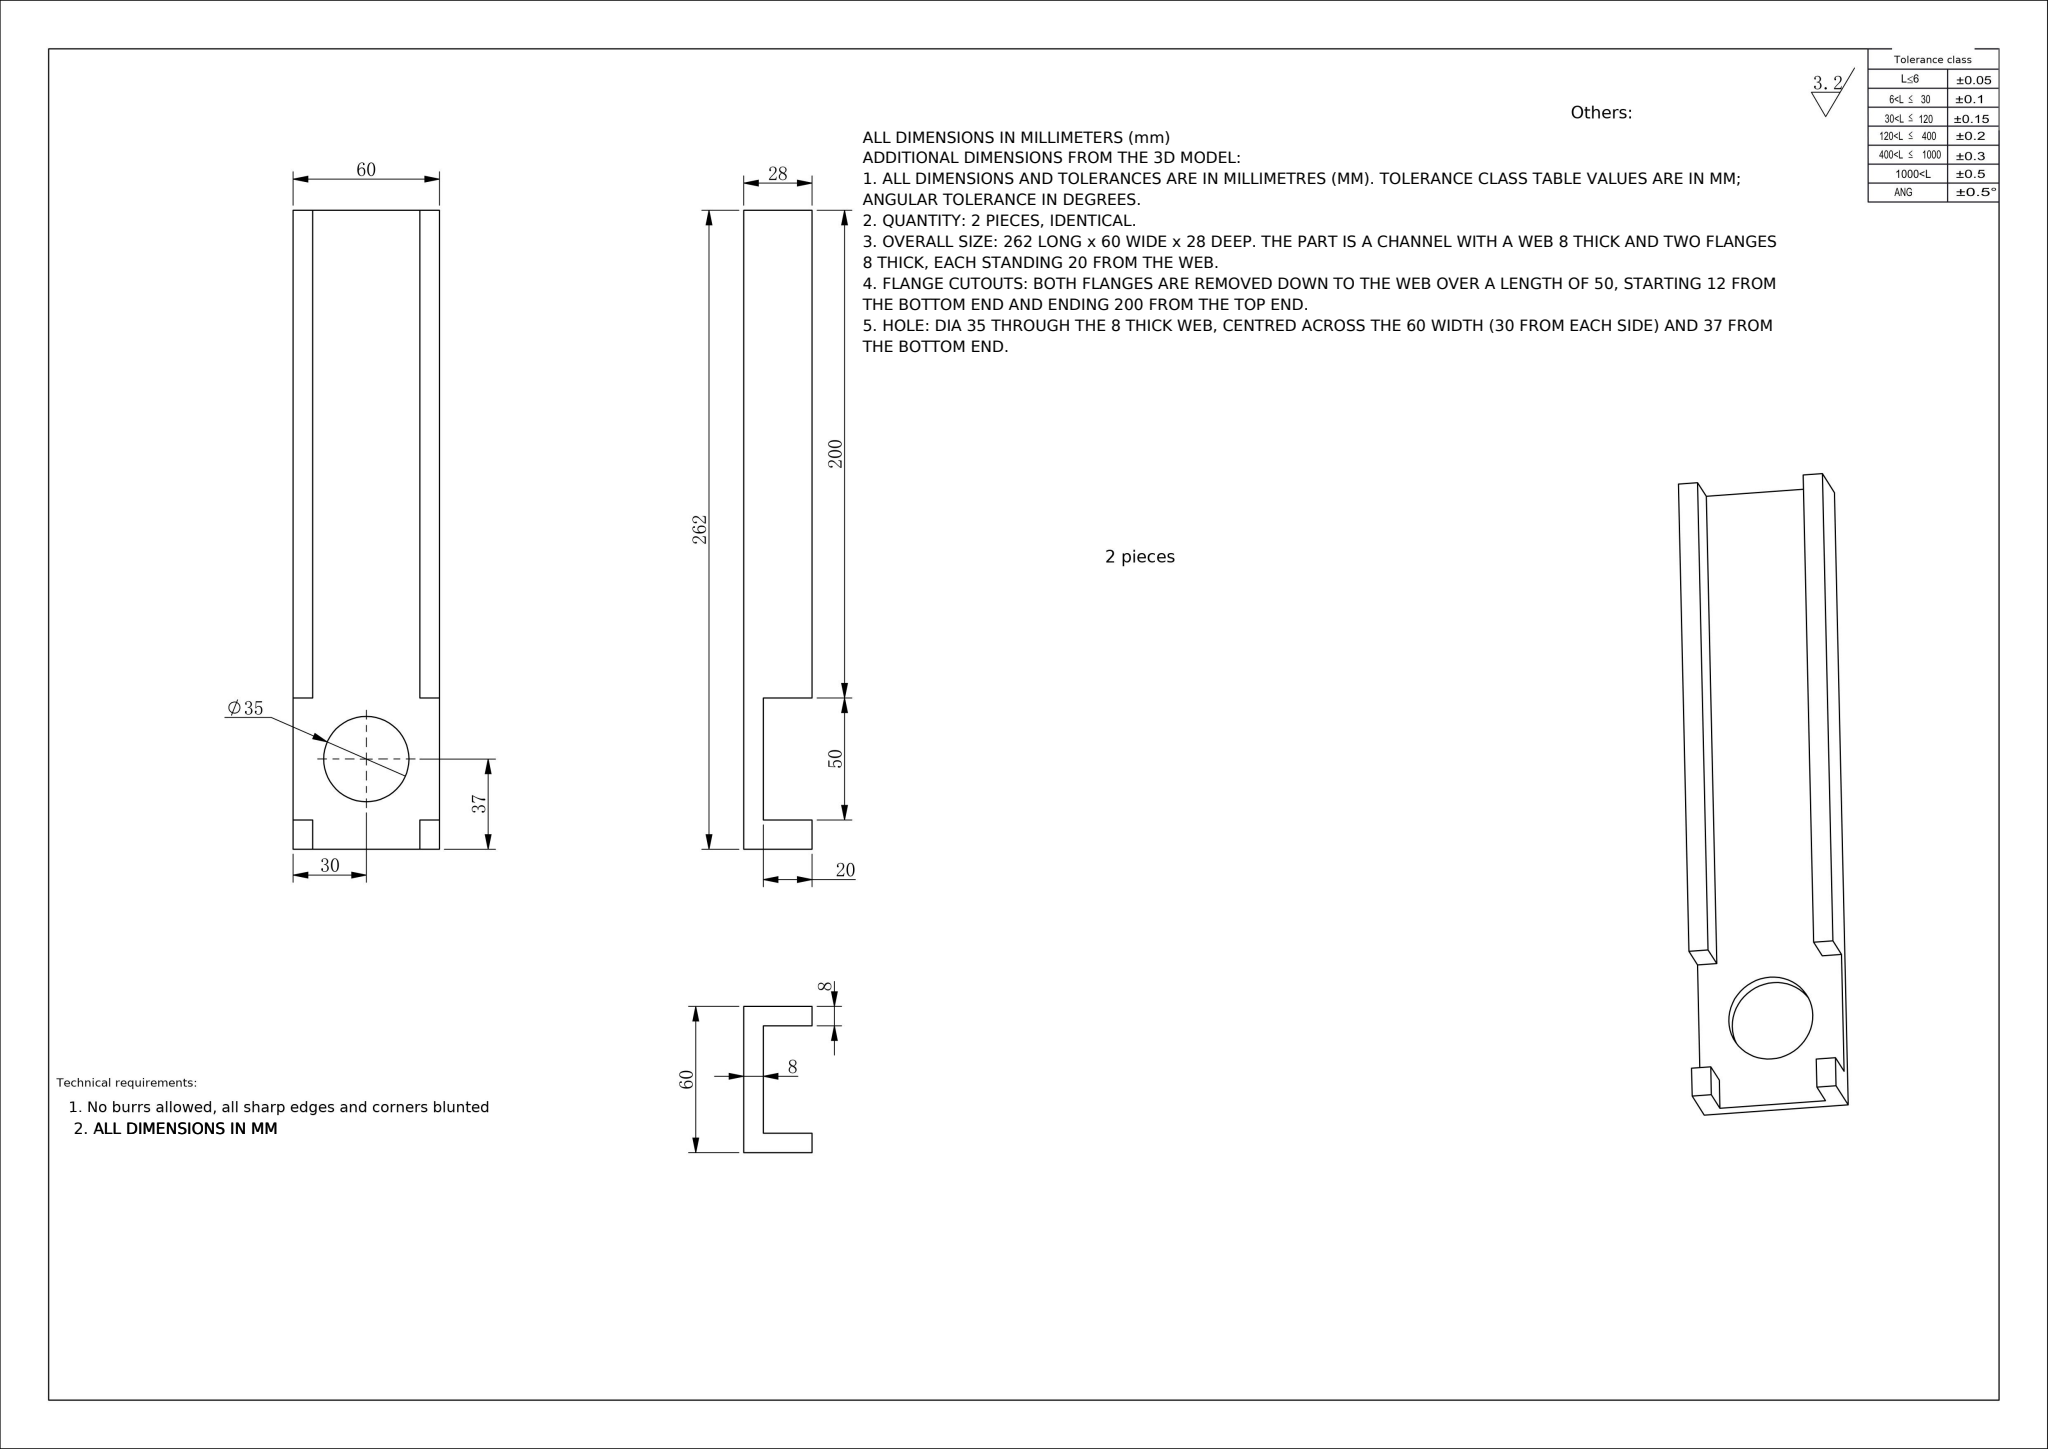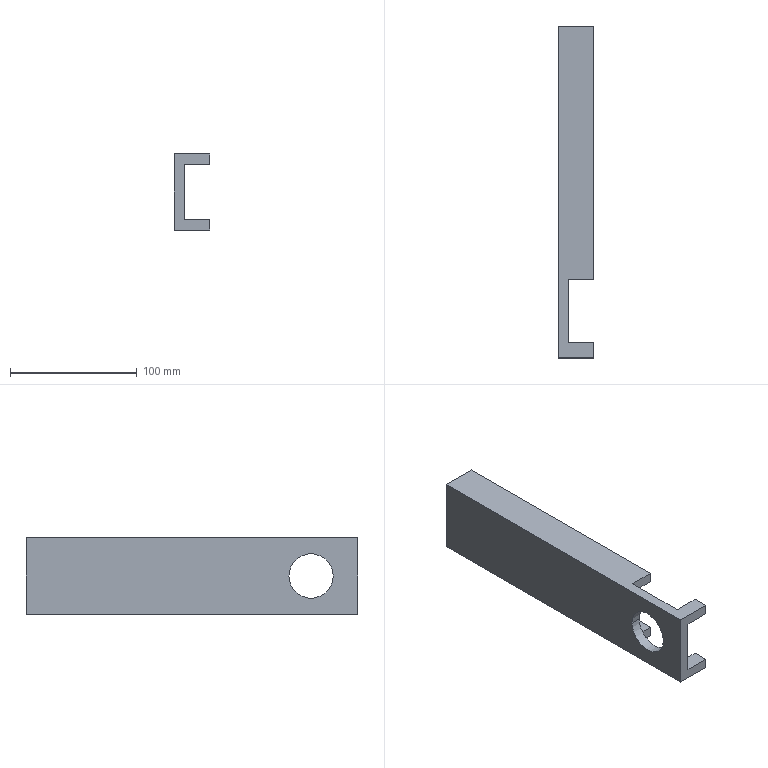Part | NX | mm | Forked Upright Pedestal Bracket | 1 solid | 20 faces | box 28 x 262 x 60 mm | volume 185903 mm3 | plane 18 | cylinder 2 | commonest cylinder face diameters 35 x2
STEP:
#1=COLOUR_RGB('',0.7922,0.8196,0.9333);
#2=FILL_AREA_STYLE_COLOUR('',#1);
#3=FILL_AREA_STYLE('',(#2));
#4=SURFACE_STYLE_FILL_AREA(#3);
#5=SURFACE_SIDE_STYLE('',(#4));
#6=SURFACE_STYLE_USAGE(.BOTH.,#5);
#7=PRESENTATION_STYLE_ASSIGNMENT((#6));
#8=CARTESIAN_POINT('',(-13.917,-176.25,22.));
#9=VERTEX_POINT('',#8);
#10=CARTESIAN_POINT('',(-13.917,-211.25,22.));
#11=VERTEX_POINT('',#10);
#12=CARTESIAN_POINT('',(-13.917,-193.75,22.));
#13=DIRECTION('',(-1.,-0.,0.));
#14=DIRECTION('',(0.,-1.,0.));
#15=AXIS2_PLACEMENT_3D('',#12,#13,#14);
#16=CIRCLE('',#15,17.5);
#17=EDGE_CURVE('',#9,#11,#16,.T.);
#18=ORIENTED_EDGE('',*,*,#17,.F.);
#19=CARTESIAN_POINT('',(-21.917,-176.25,22.));
#20=VERTEX_POINT('',#19);
#21=CARTESIAN_POINT('',(6.083,-176.25,22.));
#22=DIRECTION('',(-1.,-0.,0.));
#23=VECTOR('',#22,1000.);
#24=LINE('',#21,#23);
#25=EDGE_CURVE('',#9,#20,#24,.T.);
#26=ORIENTED_EDGE('',*,*,#25,.T.);
#27=CARTESIAN_POINT('',(-21.917,-211.25,22.));
#28=VERTEX_POINT('',#27);
#29=CARTESIAN_POINT('',(-21.917,-193.75,22.));
#30=DIRECTION('',(-1.,-0.,0.));
#31=DIRECTION('',(0.,-1.,0.));
#32=AXIS2_PLACEMENT_3D('',#29,#30,#31);
#33=CIRCLE('',#32,17.5);
#34=EDGE_CURVE('',#20,#28,#33,.T.);
#35=ORIENTED_EDGE('',*,*,#34,.T.);
#36=CARTESIAN_POINT('',(6.083,-211.25,22.));
#37=DIRECTION('',(-1.,-0.,0.));
#38=VECTOR('',#37,1000.);
#39=LINE('',#36,#38);
#40=EDGE_CURVE('',#11,#28,#39,.T.);
#41=ORIENTED_EDGE('',*,*,#40,.F.);
#42=EDGE_LOOP('',(#18,#26,#35,#41));
#43=FACE_OUTER_BOUND('',#42,.T.);
#44=CARTESIAN_POINT('',(6.083,-193.75,22.));
#45=DIRECTION('',(-1.,-0.,0.));
#46=DIRECTION('',(0.,-1.,0.));
#47=AXIS2_PLACEMENT_3D('',#44,#45,#46);
#48=CYLINDRICAL_SURFACE('',#47,17.5);
#49=ADVANCED_FACE('',(#43),#48,.F.);
#50=CARTESIAN_POINT('',(-13.917,-168.75,0.));
#51=VERTEX_POINT('',#50);
#52=CARTESIAN_POINT('',(-13.917,31.25,0.));
#53=VERTEX_POINT('',#52);
#54=CARTESIAN_POINT('',(-13.917,31.25,0.));
#55=DIRECTION('',(-0.,1.,0.));
#56=VECTOR('',#55,1000.);
#57=LINE('',#54,#56);
#58=EDGE_CURVE('',#51,#53,#57,.T.);
#59=ORIENTED_EDGE('',*,*,#58,.F.);
#60=CARTESIAN_POINT('',(6.083,-168.75,0.));
#61=VERTEX_POINT('',#60);
#62=CARTESIAN_POINT('',(6.083,-168.75,0.));
#63=DIRECTION('',(1.,0.,0.));
#64=VECTOR('',#63,1000.);
#65=LINE('',#62,#64);
#66=EDGE_CURVE('',#51,#61,#65,.T.);
#67=ORIENTED_EDGE('',*,*,#66,.T.);
#68=CARTESIAN_POINT('',(6.083,31.25,0.));
#69=VERTEX_POINT('',#68);
#70=CARTESIAN_POINT('',(6.083,31.25,0.));
#71=DIRECTION('',(0.,-1.,0.));
#72=VECTOR('',#71,1000.);
#73=LINE('',#70,#72);
#74=EDGE_CURVE('',#69,#61,#73,.T.);
#75=ORIENTED_EDGE('',*,*,#74,.F.);
#76=CARTESIAN_POINT('',(6.083,31.25,0.));
#77=DIRECTION('',(-1.,-0.,0.));
#78=VECTOR('',#77,1000.);
#79=LINE('',#76,#78);
#80=EDGE_CURVE('',#69,#53,#79,.T.);
#81=ORIENTED_EDGE('',*,*,#80,.T.);
#82=EDGE_LOOP('',(#59,#67,#75,#81));
#83=FACE_OUTER_BOUND('',#82,.T.);
#84=CARTESIAN_POINT('',(6.083,31.25,0.));
#85=DIRECTION('',(0.,0.,-1.));
#86=DIRECTION('',(-1.,0.,0.));
#87=AXIS2_PLACEMENT_3D('',#84,#85,#86);
#88=PLANE('',#87);
#89=ADVANCED_FACE('',(#83),#88,.F.);
#90=ORIENTED_EDGE('',*,*,#74,.T.);
#91=CARTESIAN_POINT('',(6.083,-168.75,-8.));
#92=VERTEX_POINT('',#91);
#93=CARTESIAN_POINT('',(6.083,-168.75,52.));
#94=DIRECTION('',(0.,0.,1.));
#95=VECTOR('',#94,1000.);
#96=LINE('',#93,#95);
#97=EDGE_CURVE('',#92,#61,#96,.T.);
#98=ORIENTED_EDGE('',*,*,#97,.F.);
#99=CARTESIAN_POINT('',(6.083,31.25,-8.));
#100=VERTEX_POINT('',#99);
#101=CARTESIAN_POINT('',(6.083,31.25,-8.));
#102=DIRECTION('',(0.,-1.,0.));
#103=VECTOR('',#102,1000.);
#104=LINE('',#101,#103);
#105=EDGE_CURVE('',#100,#92,#104,.T.);
#106=ORIENTED_EDGE('',*,*,#105,.F.);
#107=CARTESIAN_POINT('',(6.083,31.25,-8.));
#108=DIRECTION('',(0.,0.,1.));
#109=VECTOR('',#108,1000.);
#110=LINE('',#107,#109);
#111=EDGE_CURVE('',#100,#69,#110,.T.);
#112=ORIENTED_EDGE('',*,*,#111,.T.);
#113=EDGE_LOOP('',(#90,#98,#106,#112));
#114=FACE_OUTER_BOUND('',#113,.T.);
#115=CARTESIAN_POINT('',(6.083,0.,0.));
#116=DIRECTION('',(-1.,-0.,0.));
#117=DIRECTION('',(0.,0.,1.));
#118=AXIS2_PLACEMENT_3D('',#115,#116,#117);
#119=PLANE('',#118);
#120=ADVANCED_FACE('',(#114),#119,.F.);
#121=CARTESIAN_POINT('',(-13.917,-168.75,44.));
#122=VERTEX_POINT('',#121);
#123=CARTESIAN_POINT('',(6.083,-168.75,44.));
#124=VERTEX_POINT('',#123);
#125=CARTESIAN_POINT('',(6.083,-168.75,44.));
#126=DIRECTION('',(1.,0.,0.));
#127=VECTOR('',#126,1000.);
#128=LINE('',#125,#127);
#129=EDGE_CURVE('',#122,#124,#128,.T.);
#130=ORIENTED_EDGE('',*,*,#129,.F.);
#131=CARTESIAN_POINT('',(-13.917,31.25,44.));
#132=VERTEX_POINT('',#131);
#133=CARTESIAN_POINT('',(-13.917,31.25,44.));
#134=DIRECTION('',(0.,-1.,0.));
#135=VECTOR('',#134,1000.);
#136=LINE('',#133,#135);
#137=EDGE_CURVE('',#132,#122,#136,.T.);
#138=ORIENTED_EDGE('',*,*,#137,.F.);
#139=CARTESIAN_POINT('',(6.083,31.25,44.));
#140=VERTEX_POINT('',#139);
#141=CARTESIAN_POINT('',(6.083,31.25,44.));
#142=DIRECTION('',(-1.,-0.,0.));
#143=VECTOR('',#142,1000.);
#144=LINE('',#141,#143);
#145=EDGE_CURVE('',#140,#132,#144,.T.);
#146=ORIENTED_EDGE('',*,*,#145,.F.);
#147=CARTESIAN_POINT('',(6.083,31.25,44.));
#148=DIRECTION('',(0.,-1.,0.));
#149=VECTOR('',#148,1000.);
#150=LINE('',#147,#149);
#151=EDGE_CURVE('',#140,#124,#150,.T.);
#152=ORIENTED_EDGE('',*,*,#151,.T.);
#153=EDGE_LOOP('',(#130,#138,#146,#152));
#154=FACE_OUTER_BOUND('',#153,.T.);
#155=CARTESIAN_POINT('',(6.083,31.25,44.));
#156=DIRECTION('',(0.,0.,-1.));
#157=DIRECTION('',(-1.,0.,0.));
#158=AXIS2_PLACEMENT_3D('',#155,#156,#157);
#159=PLANE('',#158);
#160=ADVANCED_FACE('',(#154),#159,.T.);
#161=CARTESIAN_POINT('',(6.083,31.25,52.));
#162=VERTEX_POINT('',#161);
#163=CARTESIAN_POINT('',(6.083,-168.75,52.));
#164=VERTEX_POINT('',#163);
#165=CARTESIAN_POINT('',(6.083,31.25,52.));
#166=DIRECTION('',(0.,-1.,0.));
#167=VECTOR('',#166,1000.);
#168=LINE('',#165,#167);
#169=EDGE_CURVE('',#162,#164,#168,.T.);
#170=ORIENTED_EDGE('',*,*,#169,.T.);
#171=CARTESIAN_POINT('',(6.083,-168.75,0.));
#172=DIRECTION('',(0.,0.,-1.));
#173=VECTOR('',#172,1000.);
#174=LINE('',#171,#173);
#175=EDGE_CURVE('',#164,#124,#174,.T.);
#176=ORIENTED_EDGE('',*,*,#175,.T.);
#177=ORIENTED_EDGE('',*,*,#151,.F.);
#178=CARTESIAN_POINT('',(6.083,31.25,44.));
#179=DIRECTION('',(0.,0.,1.));
#180=VECTOR('',#179,1000.);
#181=LINE('',#178,#180);
#182=EDGE_CURVE('',#140,#162,#181,.T.);
#183=ORIENTED_EDGE('',*,*,#182,.T.);
#184=EDGE_LOOP('',(#170,#176,#177,#183));
#185=FACE_OUTER_BOUND('',#184,.T.);
#186=CARTESIAN_POINT('',(6.083,0.,0.));
#187=DIRECTION('',(-1.,-0.,0.));
#188=DIRECTION('',(0.,0.,1.));
#189=AXIS2_PLACEMENT_3D('',#186,#187,#188);
#190=PLANE('',#189);
#191=ADVANCED_FACE('',(#185),#190,.F.);
#192=CARTESIAN_POINT('',(-21.917,-193.75,22.));
#193=DIRECTION('',(-1.,-0.,0.));
#194=DIRECTION('',(0.,-1.,0.));
#195=AXIS2_PLACEMENT_3D('',#192,#193,#194);
#196=CIRCLE('',#195,17.5);
#197=EDGE_CURVE('',#28,#20,#196,.T.);
#198=ORIENTED_EDGE('',*,*,#197,.F.);
#199=ORIENTED_EDGE('',*,*,#34,.F.);
#200=EDGE_LOOP('',(#198,#199));
#201=FACE_BOUND('',#200,.T.);
#202=CARTESIAN_POINT('',(-21.917,31.25,-8.));
#203=VERTEX_POINT('',#202);
#204=CARTESIAN_POINT('',(-21.917,-230.75,-8.));
#205=VERTEX_POINT('',#204);
#206=CARTESIAN_POINT('',(-21.917,31.25,-8.));
#207=DIRECTION('',(0.,-1.,0.));
#208=VECTOR('',#207,1000.);
#209=LINE('',#206,#208);
#210=EDGE_CURVE('',#203,#205,#209,.T.);
#211=ORIENTED_EDGE('',*,*,#210,.T.);
#212=CARTESIAN_POINT('',(-21.917,-230.75,52.));
#213=VERTEX_POINT('',#212);
#214=CARTESIAN_POINT('',(-21.917,-230.75,52.));
#215=DIRECTION('',(0.,0.,-1.));
#216=VECTOR('',#215,1000.);
#217=LINE('',#214,#216);
#218=EDGE_CURVE('',#213,#205,#217,.T.);
#219=ORIENTED_EDGE('',*,*,#218,.F.);
#220=CARTESIAN_POINT('',(-21.917,31.25,52.));
#221=VERTEX_POINT('',#220);
#222=CARTESIAN_POINT('',(-21.917,31.25,52.));
#223=DIRECTION('',(0.,-1.,0.));
#224=VECTOR('',#223,1000.);
#225=LINE('',#222,#224);
#226=EDGE_CURVE('',#221,#213,#225,.T.);
#227=ORIENTED_EDGE('',*,*,#226,.F.);
#228=CARTESIAN_POINT('',(-21.917,31.25,52.));
#229=DIRECTION('',(0.,0.,-1.));
#230=VECTOR('',#229,1000.);
#231=LINE('',#228,#230);
#232=EDGE_CURVE('',#221,#203,#231,.T.);
#233=ORIENTED_EDGE('',*,*,#232,.T.);
#234=EDGE_LOOP('',(#211,#219,#227,#233));
#235=FACE_OUTER_BOUND('',#234,.T.);
#236=CARTESIAN_POINT('',(-21.917,31.25,52.));
#237=DIRECTION('',(1.,0.,0.));
#238=DIRECTION('',(-0.,1.,0.));
#239=AXIS2_PLACEMENT_3D('',#236,#237,#238);
#240=PLANE('',#239);
#241=ADVANCED_FACE('',(#201,#235),#240,.F.);
#242=CARTESIAN_POINT('',(-13.917,-230.75,44.));
#243=VERTEX_POINT('',#242);
#244=CARTESIAN_POINT('',(-13.917,-230.75,0.));
#245=VERTEX_POINT('',#244);
#246=CARTESIAN_POINT('',(-13.917,-230.75,52.));
#247=DIRECTION('',(0.,0.,-1.));
#248=VECTOR('',#247,1000.);
#249=LINE('',#246,#248);
#250=EDGE_CURVE('',#243,#245,#249,.T.);
#251=ORIENTED_EDGE('',*,*,#250,.F.);
#252=CARTESIAN_POINT('',(6.083,-230.75,44.));
#253=VERTEX_POINT('',#252);
#254=CARTESIAN_POINT('',(6.083,-230.75,44.));
#255=DIRECTION('',(-1.,-0.,0.));
#256=VECTOR('',#255,1000.);
#257=LINE('',#254,#256);
#258=EDGE_CURVE('',#253,#243,#257,.T.);
#259=ORIENTED_EDGE('',*,*,#258,.F.);
#260=CARTESIAN_POINT('',(6.083,-230.75,52.));
#261=VERTEX_POINT('',#260);
#262=CARTESIAN_POINT('',(6.083,-230.75,52.));
#263=DIRECTION('',(0.,0.,-1.));
#264=VECTOR('',#263,1000.);
#265=LINE('',#262,#264);
#266=EDGE_CURVE('',#261,#253,#265,.T.);
#267=ORIENTED_EDGE('',*,*,#266,.F.);
#268=CARTESIAN_POINT('',(-21.917,-230.75,52.));
#269=DIRECTION('',(1.,0.,0.));
#270=VECTOR('',#269,1000.);
#271=LINE('',#268,#270);
#272=EDGE_CURVE('',#213,#261,#271,.T.);
#273=ORIENTED_EDGE('',*,*,#272,.F.);
#274=ORIENTED_EDGE('',*,*,#218,.T.);
#275=CARTESIAN_POINT('',(6.083,-230.75,-8.));
#276=VERTEX_POINT('',#275);
#277=CARTESIAN_POINT('',(6.083,-230.75,-8.));
#278=DIRECTION('',(-1.,-0.,0.));
#279=VECTOR('',#278,1000.);
#280=LINE('',#277,#279);
#281=EDGE_CURVE('',#276,#205,#280,.T.);
#282=ORIENTED_EDGE('',*,*,#281,.F.);
#283=CARTESIAN_POINT('',(6.083,-230.75,0.));
#284=VERTEX_POINT('',#283);
#285=CARTESIAN_POINT('',(6.083,-230.75,0.));
#286=DIRECTION('',(0.,0.,-1.));
#287=VECTOR('',#286,1000.);
#288=LINE('',#285,#287);
#289=EDGE_CURVE('',#284,#276,#288,.T.);
#290=ORIENTED_EDGE('',*,*,#289,.F.);
#291=CARTESIAN_POINT('',(6.083,-230.75,0.));
#292=DIRECTION('',(-1.,-0.,0.));
#293=VECTOR('',#292,1000.);
#294=LINE('',#291,#293);
#295=EDGE_CURVE('',#284,#245,#294,.T.);
#296=ORIENTED_EDGE('',*,*,#295,.T.);
#297=EDGE_LOOP('',(#251,#259,#267,#273,#274,#282,#290,#296));
#298=FACE_OUTER_BOUND('',#297,.T.);
#299=CARTESIAN_POINT('',(-21.917,-230.75,52.));
#300=DIRECTION('',(0.,1.,0.));
#301=DIRECTION('',(0.,0.,1.));
#302=AXIS2_PLACEMENT_3D('',#299,#300,#301);
#303=PLANE('',#302);
#304=ADVANCED_FACE('',(#298),#303,.F.);
#305=CARTESIAN_POINT('',(-13.917,-218.75,0.));
#306=VERTEX_POINT('',#305);
#307=CARTESIAN_POINT('',(-13.917,31.25,0.));
#308=DIRECTION('',(-0.,1.,0.));
#309=VECTOR('',#308,1000.);
#310=LINE('',#307,#309);
#311=EDGE_CURVE('',#245,#306,#310,.T.);
#312=ORIENTED_EDGE('',*,*,#311,.T.);
#313=CARTESIAN_POINT('',(-13.917,-218.75,-8.));
#314=VERTEX_POINT('',#313);
#315=CARTESIAN_POINT('',(-13.917,-218.75,52.));
#316=DIRECTION('',(0.,0.,-1.));
#317=VECTOR('',#316,1000.);
#318=LINE('',#315,#317);
#319=EDGE_CURVE('',#306,#314,#318,.T.);
#320=ORIENTED_EDGE('',*,*,#319,.T.);
#321=CARTESIAN_POINT('',(-13.917,-168.75,-8.));
#322=VERTEX_POINT('',#321);
#323=CARTESIAN_POINT('',(-13.917,-168.75,-8.));
#324=DIRECTION('',(-0.,1.,-0.));
#325=VECTOR('',#324,1000.);
#326=LINE('',#323,#325);
#327=EDGE_CURVE('',#314,#322,#326,.T.);
#328=ORIENTED_EDGE('',*,*,#327,.T.);
#329=CARTESIAN_POINT('',(-13.917,-168.75,52.));
#330=DIRECTION('',(0.,0.,1.));
#331=VECTOR('',#330,1000.);
#332=LINE('',#329,#331);
#333=EDGE_CURVE('',#322,#51,#332,.T.);
#334=ORIENTED_EDGE('',*,*,#333,.T.);
#335=ORIENTED_EDGE('',*,*,#58,.T.);
#336=CARTESIAN_POINT('',(-13.917,31.25,52.));
#337=DIRECTION('',(0.,0.,-1.));
#338=VECTOR('',#337,1000.);
#339=LINE('',#336,#338);
#340=EDGE_CURVE('',#132,#53,#339,.T.);
#341=ORIENTED_EDGE('',*,*,#340,.F.);
#342=ORIENTED_EDGE('',*,*,#137,.T.);
#343=CARTESIAN_POINT('',(-13.917,-168.75,52.));
#344=VERTEX_POINT('',#343);
#345=CARTESIAN_POINT('',(-13.917,-168.75,52.));
#346=DIRECTION('',(0.,0.,1.));
#347=VECTOR('',#346,1000.);
#348=LINE('',#345,#347);
#349=EDGE_CURVE('',#122,#344,#348,.T.);
#350=ORIENTED_EDGE('',*,*,#349,.T.);
#351=CARTESIAN_POINT('',(-13.917,-218.75,52.));
#352=VERTEX_POINT('',#351);
#353=CARTESIAN_POINT('',(-13.917,-168.75,52.));
#354=DIRECTION('',(0.,-1.,-0.));
#355=VECTOR('',#354,1000.);
#356=LINE('',#353,#355);
#357=EDGE_CURVE('',#344,#352,#356,.T.);
#358=ORIENTED_EDGE('',*,*,#357,.T.);
#359=CARTESIAN_POINT('',(-13.917,-218.75,44.));
#360=VERTEX_POINT('',#359);
#361=CARTESIAN_POINT('',(-13.917,-218.75,52.));
#362=DIRECTION('',(0.,0.,-1.));
#363=VECTOR('',#362,1000.);
#364=LINE('',#361,#363);
#365=EDGE_CURVE('',#352,#360,#364,.T.);
#366=ORIENTED_EDGE('',*,*,#365,.T.);
#367=CARTESIAN_POINT('',(-13.917,31.25,44.));
#368=DIRECTION('',(0.,-1.,0.));
#369=VECTOR('',#368,1000.);
#370=LINE('',#367,#369);
#371=EDGE_CURVE('',#360,#243,#370,.T.);
#372=ORIENTED_EDGE('',*,*,#371,.T.);
#373=ORIENTED_EDGE('',*,*,#250,.T.);
#374=EDGE_LOOP('',(#312,#320,#328,#334,#335,#341,#342,#350,#358,#366,#372,#373));
#375=FACE_OUTER_BOUND('',#374,.T.);
#376=CARTESIAN_POINT('',(-13.917,-193.75,22.));
#377=DIRECTION('',(-1.,-0.,0.));
#378=DIRECTION('',(0.,-1.,0.));
#379=AXIS2_PLACEMENT_3D('',#376,#377,#378);
#380=CIRCLE('',#379,17.5);
#381=EDGE_CURVE('',#11,#9,#380,.T.);
#382=ORIENTED_EDGE('',*,*,#381,.T.);
#383=ORIENTED_EDGE('',*,*,#17,.T.);
#384=EDGE_LOOP('',(#382,#383));
#385=FACE_BOUND('',#384,.T.);
#386=CARTESIAN_POINT('',(-13.917,31.25,52.));
#387=DIRECTION('',(-1.,-0.,0.));
#388=DIRECTION('',(0.,-1.,0.));
#389=AXIS2_PLACEMENT_3D('',#386,#387,#388);
#390=PLANE('',#389);
#391=ADVANCED_FACE('',(#375,#385),#390,.F.);
#392=CARTESIAN_POINT('',(6.083,31.25,-8.));
#393=DIRECTION('',(-1.,-0.,0.));
#394=VECTOR('',#393,1000.);
#395=LINE('',#392,#394);
#396=EDGE_CURVE('',#100,#203,#395,.T.);
#397=ORIENTED_EDGE('',*,*,#396,.T.);
#398=ORIENTED_EDGE('',*,*,#232,.F.);
#399=CARTESIAN_POINT('',(-21.917,31.25,52.));
#400=DIRECTION('',(-1.,0.,0.));
#401=VECTOR('',#400,1000.);
#402=LINE('',#399,#401);
#403=EDGE_CURVE('',#162,#221,#402,.T.);
#404=ORIENTED_EDGE('',*,*,#403,.F.);
#405=ORIENTED_EDGE('',*,*,#182,.F.);
#406=ORIENTED_EDGE('',*,*,#145,.T.);
#407=ORIENTED_EDGE('',*,*,#340,.T.);
#408=ORIENTED_EDGE('',*,*,#80,.F.);
#409=ORIENTED_EDGE('',*,*,#111,.F.);
#410=EDGE_LOOP('',(#397,#398,#404,#405,#406,#407,#408,#409));
#411=FACE_OUTER_BOUND('',#410,.T.);
#412=CARTESIAN_POINT('',(-21.917,31.25,52.));
#413=DIRECTION('',(0.,-1.,0.));
#414=DIRECTION('',(0.,0.,-1.));
#415=AXIS2_PLACEMENT_3D('',#412,#413,#414);
#416=PLANE('',#415);
#417=ADVANCED_FACE('',(#411),#416,.F.);
#418=CARTESIAN_POINT('',(-13.917,-168.75,52.));
#419=DIRECTION('',(1.,0.,0.));
#420=VECTOR('',#419,1000.);
#421=LINE('',#418,#420);
#422=EDGE_CURVE('',#344,#164,#421,.T.);
#423=ORIENTED_EDGE('',*,*,#422,.T.);
#424=ORIENTED_EDGE('',*,*,#169,.F.);
#425=ORIENTED_EDGE('',*,*,#403,.T.);
#426=ORIENTED_EDGE('',*,*,#226,.T.);
#427=ORIENTED_EDGE('',*,*,#272,.T.);
#428=CARTESIAN_POINT('',(6.083,-218.75,52.));
#429=VERTEX_POINT('',#428);
#430=CARTESIAN_POINT('',(6.083,31.25,52.));
#431=DIRECTION('',(0.,-1.,0.));
#432=VECTOR('',#431,1000.);
#433=LINE('',#430,#432);
#434=EDGE_CURVE('',#429,#261,#433,.T.);
#435=ORIENTED_EDGE('',*,*,#434,.F.);
#436=CARTESIAN_POINT('',(-13.917,-218.75,52.));
#437=DIRECTION('',(1.,0.,0.));
#438=VECTOR('',#437,1000.);
#439=LINE('',#436,#438);
#440=EDGE_CURVE('',#352,#429,#439,.T.);
#441=ORIENTED_EDGE('',*,*,#440,.F.);
#442=ORIENTED_EDGE('',*,*,#357,.F.);
#443=EDGE_LOOP('',(#423,#424,#425,#426,#427,#435,#441,#442));
#444=FACE_OUTER_BOUND('',#443,.T.);
#445=CARTESIAN_POINT('',(0.,0.,52.));
#446=DIRECTION('',(0.,0.,1.));
#447=DIRECTION('',(1.,0.,0.));
#448=AXIS2_PLACEMENT_3D('',#445,#446,#447);
#449=PLANE('',#448);
#450=ADVANCED_FACE('',(#444),#449,.T.);
#451=CARTESIAN_POINT('',(-13.917,-168.75,-8.));
#452=DIRECTION('',(1.,0.,0.));
#453=VECTOR('',#452,1000.);
#454=LINE('',#451,#453);
#455=EDGE_CURVE('',#322,#92,#454,.T.);
#456=ORIENTED_EDGE('',*,*,#455,.F.);
#457=ORIENTED_EDGE('',*,*,#327,.F.);
#458=CARTESIAN_POINT('',(6.083,-218.75,-8.));
#459=VERTEX_POINT('',#458);
#460=CARTESIAN_POINT('',(-13.917,-218.75,-8.));
#461=DIRECTION('',(1.,0.,0.));
#462=VECTOR('',#461,1000.);
#463=LINE('',#460,#462);
#464=EDGE_CURVE('',#314,#459,#463,.T.);
#465=ORIENTED_EDGE('',*,*,#464,.T.);
#466=CARTESIAN_POINT('',(6.083,31.25,-8.));
#467=DIRECTION('',(0.,-1.,0.));
#468=VECTOR('',#467,1000.);
#469=LINE('',#466,#468);
#470=EDGE_CURVE('',#459,#276,#469,.T.);
#471=ORIENTED_EDGE('',*,*,#470,.T.);
#472=ORIENTED_EDGE('',*,*,#281,.T.);
#473=ORIENTED_EDGE('',*,*,#210,.F.);
#474=ORIENTED_EDGE('',*,*,#396,.F.);
#475=ORIENTED_EDGE('',*,*,#105,.T.);
#476=EDGE_LOOP('',(#456,#457,#465,#471,#472,#473,#474,#475));
#477=FACE_OUTER_BOUND('',#476,.T.);
#478=CARTESIAN_POINT('',(6.083,31.25,-8.));
#479=DIRECTION('',(0.,0.,-1.));
#480=DIRECTION('',(-1.,0.,0.));
#481=AXIS2_PLACEMENT_3D('',#478,#479,#480);
#482=PLANE('',#481);
#483=ADVANCED_FACE('',(#477),#482,.T.);
#484=CARTESIAN_POINT('',(6.083,-218.75,0.));
#485=VERTEX_POINT('',#484);
#486=CARTESIAN_POINT('',(6.083,31.25,0.));
#487=DIRECTION('',(0.,-1.,0.));
#488=VECTOR('',#487,1000.);
#489=LINE('',#486,#488);
#490=EDGE_CURVE('',#485,#284,#489,.T.);
#491=ORIENTED_EDGE('',*,*,#490,.F.);
#492=CARTESIAN_POINT('',(6.083,-218.75,0.));
#493=DIRECTION('',(-1.,-0.,0.));
#494=VECTOR('',#493,1000.);
#495=LINE('',#492,#494);
#496=EDGE_CURVE('',#485,#306,#495,.T.);
#497=ORIENTED_EDGE('',*,*,#496,.T.);
#498=ORIENTED_EDGE('',*,*,#311,.F.);
#499=ORIENTED_EDGE('',*,*,#295,.F.);
#500=EDGE_LOOP('',(#491,#497,#498,#499));
#501=FACE_OUTER_BOUND('',#500,.T.);
#502=CARTESIAN_POINT('',(6.083,31.25,0.));
#503=DIRECTION('',(0.,0.,-1.));
#504=DIRECTION('',(-1.,0.,0.));
#505=AXIS2_PLACEMENT_3D('',#502,#503,#504);
#506=PLANE('',#505);
#507=ADVANCED_FACE('',(#501),#506,.F.);
#508=ORIENTED_EDGE('',*,*,#470,.F.);
#509=CARTESIAN_POINT('',(6.083,-218.75,52.));
#510=DIRECTION('',(0.,0.,-1.));
#511=VECTOR('',#510,1000.);
#512=LINE('',#509,#511);
#513=EDGE_CURVE('',#485,#459,#512,.T.);
#514=ORIENTED_EDGE('',*,*,#513,.F.);
#515=ORIENTED_EDGE('',*,*,#490,.T.);
#516=ORIENTED_EDGE('',*,*,#289,.T.);
#517=EDGE_LOOP('',(#508,#514,#515,#516));
#518=FACE_OUTER_BOUND('',#517,.T.);
#519=CARTESIAN_POINT('',(6.083,0.,0.));
#520=DIRECTION('',(-1.,-0.,0.));
#521=DIRECTION('',(0.,0.,1.));
#522=AXIS2_PLACEMENT_3D('',#519,#520,#521);
#523=PLANE('',#522);
#524=ADVANCED_FACE('',(#518),#523,.F.);
#525=CARTESIAN_POINT('',(6.083,-218.75,44.));
#526=VERTEX_POINT('',#525);
#527=CARTESIAN_POINT('',(6.083,-218.75,44.));
#528=DIRECTION('',(-1.,-0.,0.));
#529=VECTOR('',#528,1000.);
#530=LINE('',#527,#529);
#531=EDGE_CURVE('',#526,#360,#530,.T.);
#532=ORIENTED_EDGE('',*,*,#531,.F.);
#533=CARTESIAN_POINT('',(6.083,31.25,44.));
#534=DIRECTION('',(0.,-1.,0.));
#535=VECTOR('',#534,1000.);
#536=LINE('',#533,#535);
#537=EDGE_CURVE('',#526,#253,#536,.T.);
#538=ORIENTED_EDGE('',*,*,#537,.T.);
#539=ORIENTED_EDGE('',*,*,#258,.T.);
#540=ORIENTED_EDGE('',*,*,#371,.F.);
#541=EDGE_LOOP('',(#532,#538,#539,#540));
#542=FACE_OUTER_BOUND('',#541,.T.);
#543=CARTESIAN_POINT('',(6.083,31.25,44.));
#544=DIRECTION('',(0.,0.,-1.));
#545=DIRECTION('',(-1.,0.,0.));
#546=AXIS2_PLACEMENT_3D('',#543,#544,#545);
#547=PLANE('',#546);
#548=ADVANCED_FACE('',(#542),#547,.T.);
#549=ORIENTED_EDGE('',*,*,#537,.F.);
#550=CARTESIAN_POINT('',(6.083,-218.75,52.));
#551=DIRECTION('',(0.,0.,-1.));
#552=VECTOR('',#551,1000.);
#553=LINE('',#550,#552);
#554=EDGE_CURVE('',#429,#526,#553,.T.);
#555=ORIENTED_EDGE('',*,*,#554,.F.);
#556=ORIENTED_EDGE('',*,*,#434,.T.);
#557=ORIENTED_EDGE('',*,*,#266,.T.);
#558=EDGE_LOOP('',(#549,#555,#556,#557));
#559=FACE_OUTER_BOUND('',#558,.T.);
#560=CARTESIAN_POINT('',(6.083,0.,0.));
#561=DIRECTION('',(-1.,-0.,0.));
#562=DIRECTION('',(0.,0.,1.));
#563=AXIS2_PLACEMENT_3D('',#560,#561,#562);
#564=PLANE('',#563);
#565=ADVANCED_FACE('',(#559),#564,.F.);
#566=ORIENTED_EDGE('',*,*,#25,.F.);
#567=ORIENTED_EDGE('',*,*,#381,.F.);
#568=ORIENTED_EDGE('',*,*,#40,.T.);
#569=ORIENTED_EDGE('',*,*,#197,.T.);
#570=EDGE_LOOP('',(#566,#567,#568,#569));
#571=FACE_OUTER_BOUND('',#570,.T.);
#572=CARTESIAN_POINT('',(6.083,-193.75,22.));
#573=DIRECTION('',(-1.,-0.,0.));
#574=DIRECTION('',(0.,-1.,0.));
#575=AXIS2_PLACEMENT_3D('',#572,#573,#574);
#576=CYLINDRICAL_SURFACE('',#575,17.5);
#577=ADVANCED_FACE('',(#571),#576,.F.);
#578=ORIENTED_EDGE('',*,*,#531,.T.);
#579=ORIENTED_EDGE('',*,*,#365,.F.);
#580=ORIENTED_EDGE('',*,*,#440,.T.);
#581=ORIENTED_EDGE('',*,*,#554,.T.);
#582=EDGE_LOOP('',(#578,#579,#580,#581));
#583=FACE_OUTER_BOUND('',#582,.T.);
#584=CARTESIAN_POINT('',(-13.917,-218.75,52.));
#585=DIRECTION('',(0.,-1.,0.));
#586=DIRECTION('',(1.,0.,0.));
#587=AXIS2_PLACEMENT_3D('',#584,#585,#586);
#588=PLANE('',#587);
#589=ADVANCED_FACE('',(#583),#588,.F.);
#590=ORIENTED_EDGE('',*,*,#129,.T.);
#591=ORIENTED_EDGE('',*,*,#175,.F.);
#592=ORIENTED_EDGE('',*,*,#422,.F.);
#593=ORIENTED_EDGE('',*,*,#349,.F.);
#594=EDGE_LOOP('',(#590,#591,#592,#593));
#595=FACE_OUTER_BOUND('',#594,.T.);
#596=CARTESIAN_POINT('',(-13.917,-168.75,52.));
#597=DIRECTION('',(-0.,1.,0.));
#598=DIRECTION('',(-1.,-0.,0.));
#599=AXIS2_PLACEMENT_3D('',#596,#597,#598);
#600=PLANE('',#599);
#601=ADVANCED_FACE('',(#595),#600,.F.);
#602=ORIENTED_EDGE('',*,*,#333,.F.);
#603=ORIENTED_EDGE('',*,*,#455,.T.);
#604=ORIENTED_EDGE('',*,*,#97,.T.);
#605=ORIENTED_EDGE('',*,*,#66,.F.);
#606=EDGE_LOOP('',(#602,#603,#604,#605));
#607=FACE_OUTER_BOUND('',#606,.T.);
#608=CARTESIAN_POINT('',(-13.917,-168.75,52.));
#609=DIRECTION('',(-0.,1.,0.));
#610=DIRECTION('',(-1.,-0.,0.));
#611=AXIS2_PLACEMENT_3D('',#608,#609,#610);
#612=PLANE('',#611);
#613=ADVANCED_FACE('',(#607),#612,.F.);
#614=ORIENTED_EDGE('',*,*,#513,.T.);
#615=ORIENTED_EDGE('',*,*,#464,.F.);
#616=ORIENTED_EDGE('',*,*,#319,.F.);
#617=ORIENTED_EDGE('',*,*,#496,.F.);
#618=EDGE_LOOP('',(#614,#615,#616,#617));
#619=FACE_OUTER_BOUND('',#618,.T.);
#620=CARTESIAN_POINT('',(-13.917,-218.75,52.));
#621=DIRECTION('',(0.,-1.,0.));
#622=DIRECTION('',(1.,0.,0.));
#623=AXIS2_PLACEMENT_3D('',#620,#621,#622);
#624=PLANE('',#623);
#625=ADVANCED_FACE('',(#619),#624,.F.);
#626=CLOSED_SHELL('',(#49,#89,#120,#160,#191,#241,#304,#391,#417,#450,#483,#507,#524,#548,#565,#577,#589,#601,#613,#625));
#627=MANIFOLD_SOLID_BREP('',#626);
#628=STYLED_ITEM('',(#7),#627);
#629=(LENGTH_UNIT()NAMED_UNIT(*)SI_UNIT(.MILLI.,.METRE.));
#630=UNCERTAINTY_MEASURE_WITH_UNIT(LENGTH_MEASURE(0.00001),#629,'','');
#631=(NAMED_UNIT(*)PLANE_ANGLE_UNIT()SI_UNIT($,.RADIAN.));
#632=(NAMED_UNIT(*)SI_UNIT($,.STERADIAN.)SOLID_ANGLE_UNIT());
#633=(GEOMETRIC_REPRESENTATION_CONTEXT(3)GLOBAL_UNCERTAINTY_ASSIGNED_CONTEXT((#630))GLOBAL_UNIT_ASSIGNED_CONTEXT((#629,#631,#632))REPRESENTATION_CONTEXT('',''));
#634=MECHANICAL_DESIGN_GEOMETRIC_PRESENTATION_REPRESENTATION('',(#628),#633);
#635=COLOUR_RGB('',0.7922,0.8196,0.9333);
#636=FILL_AREA_STYLE_COLOUR('',#635);
#637=FILL_AREA_STYLE('',(#636));
#638=SURFACE_STYLE_FILL_AREA(#637);
#639=SURFACE_SIDE_STYLE('',(#638));
#640=SURFACE_STYLE_USAGE(.BOTH.,#639);
#641=PRESENTATION_STYLE_ASSIGNMENT((#640));
#642=CARTESIAN_POINT('',(0.,0.,0.));
#643=DIRECTION('',(0.,0.,1.));
#644=DIRECTION('',(1.,0.,0.));
#645=AXIS2_PLACEMENT_3D('',#642,#643,#644);
#646=(LENGTH_UNIT()NAMED_UNIT(*)SI_UNIT(.MILLI.,.METRE.));
#647=UNCERTAINTY_MEASURE_WITH_UNIT(LENGTH_MEASURE(0.00001),#646,'','');
#648=(NAMED_UNIT(*)PLANE_ANGLE_UNIT()SI_UNIT($,.RADIAN.));
#649=(NAMED_UNIT(*)SI_UNIT($,.STERADIAN.)SOLID_ANGLE_UNIT());
#650=(GEOMETRIC_REPRESENTATION_CONTEXT(3)GLOBAL_UNCERTAINTY_ASSIGNED_CONTEXT((#647))GLOBAL_UNIT_ASSIGNED_CONTEXT((#646,#648,#649))REPRESENTATION_CONTEXT('',''));
#651=ADVANCED_BREP_SHAPE_REPRESENTATION('',(#627,#645),#650);
#652=STYLED_ITEM('',(#641),#651);
#653=PRESENTATION_LAYER_ASSIGNMENT('','',(#652));
#654=PRESENTATION_LAYER_ASSIGNMENT('','',(#628));
#655=(LENGTH_UNIT()NAMED_UNIT(*)SI_UNIT(.MILLI.,.METRE.));
#656=UNCERTAINTY_MEASURE_WITH_UNIT(LENGTH_MEASURE(0.00001),#655,'','');
#657=(NAMED_UNIT(*)PLANE_ANGLE_UNIT()SI_UNIT($,.RADIAN.));
#658=(NAMED_UNIT(*)SI_UNIT($,.STERADIAN.)SOLID_ANGLE_UNIT());
#659=(GEOMETRIC_REPRESENTATION_CONTEXT(3)GLOBAL_UNCERTAINTY_ASSIGNED_CONTEXT((#656))GLOBAL_UNIT_ASSIGNED_CONTEXT((#655,#657,#658))REPRESENTATION_CONTEXT('',''));
#660=MECHANICAL_DESIGN_GEOMETRIC_PRESENTATION_REPRESENTATION('',(#652),#659);